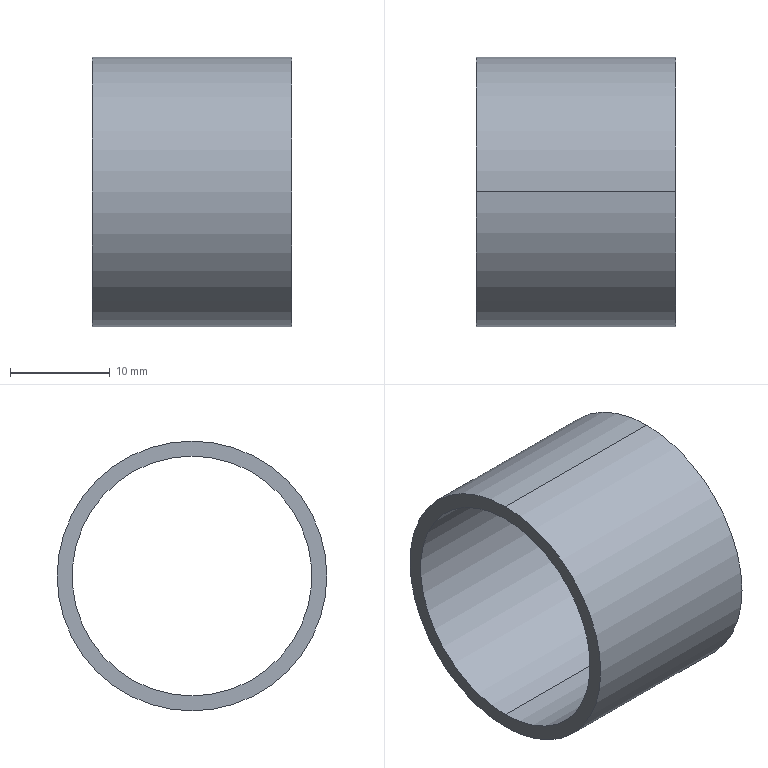Component | SolidWorks | ClampingAssembly-2_CopperSleeve24X27X10-2 | 1 solid | 6 faces | box 20 x 27 x 27 mm | volume 2403 mm3 | cylinder 4 | plane 2 | commonest cylinder face diameters 24 x2 27 x2 | material Bronze Bronze
build123d program:
from build123d import *

# Parameters (mm, degrees)
SKETCH1_R           = 13.5
SKETCH1_R_2         = 12
BOSS_EXTRUDE1_DEPTH = 20


with BuildPart() as part:
    # Sketch1 → Boss-Extrude1 (new body)
    with BuildSketch(Plane.XY):
        Circle(SKETCH1_R)
        Circle(SKETCH1_R_2, mode=Mode.SUBTRACT)
    extrude(amount=BOSS_EXTRUDE1_DEPTH)


solid = part.part

# Placed as in the assembly
solid = solid.moved(Location((-173.215, -74.917, -1210.457), (0, 90, 0)))
STEP:
#1=COLOUR_RGB('',0.7922,0.8196,0.9333);
#2=FILL_AREA_STYLE_COLOUR('',#1);
#3=FILL_AREA_STYLE('',(#2));
#4=SURFACE_STYLE_FILL_AREA(#3);
#5=SURFACE_SIDE_STYLE('',(#4));
#6=SURFACE_STYLE_USAGE(.BOTH.,#5);
#7=PRESENTATION_STYLE_ASSIGNMENT((#6));
#8=CARTESIAN_POINT('',(-6.819,-2.949,-47.183));
#9=VERTEX_POINT('',#8);
#10=CARTESIAN_POINT('',(-6.819,-2.949,-48.128));
#11=VERTEX_POINT('',#10);
#12=CARTESIAN_POINT('',(-6.819,-2.949,-47.656));
#13=DIRECTION('',(-1.,0.,-0.));
#14=DIRECTION('',(0.,0.,-1.));
#15=AXIS2_PLACEMENT_3D('',#12,#13,#14);
#16=CIRCLE('',#15,0.4724);
#17=EDGE_CURVE('',#9,#11,#16,.T.);
#18=ORIENTED_EDGE('',*,*,#17,.T.);
#19=CARTESIAN_POINT('',(-6.032,-2.949,-48.128));
#20=VERTEX_POINT('',#19);
#21=CARTESIAN_POINT('',(-6.819,-2.949,-48.128));
#22=DIRECTION('',(1.,-0.,0.));
#23=VECTOR('',#22,39.37);
#24=LINE('',#21,#23);
#25=EDGE_CURVE('',#11,#20,#24,.T.);
#26=ORIENTED_EDGE('',*,*,#25,.T.);
#27=CARTESIAN_POINT('',(-6.032,-2.949,-47.183));
#28=VERTEX_POINT('',#27);
#29=CARTESIAN_POINT('',(-6.032,-2.949,-47.656));
#30=DIRECTION('',(-1.,0.,-0.));
#31=DIRECTION('',(0.,0.,-1.));
#32=AXIS2_PLACEMENT_3D('',#29,#30,#31);
#33=CIRCLE('',#32,0.4724);
#34=EDGE_CURVE('',#28,#20,#33,.T.);
#35=ORIENTED_EDGE('',*,*,#34,.F.);
#36=CARTESIAN_POINT('',(-6.819,-2.949,-47.183));
#37=DIRECTION('',(1.,-0.,0.));
#38=VECTOR('',#37,39.37);
#39=LINE('',#36,#38);
#40=EDGE_CURVE('',#9,#28,#39,.T.);
#41=ORIENTED_EDGE('',*,*,#40,.F.);
#42=EDGE_LOOP('',(#18,#26,#35,#41));
#43=FACE_OUTER_BOUND('',#42,.T.);
#44=CARTESIAN_POINT('',(-6.819,-2.949,-47.656));
#45=DIRECTION('',(1.,-0.,0.));
#46=DIRECTION('',(0.,-0.,1.));
#47=AXIS2_PLACEMENT_3D('',#44,#45,#46);
#48=CYLINDRICAL_SURFACE('',#47,0.4724);
#49=ADVANCED_FACE('',(#43),#48,.F.);
#50=CARTESIAN_POINT('',(-6.819,-2.949,-48.187));
#51=VERTEX_POINT('',#50);
#52=CARTESIAN_POINT('',(-6.819,-2.949,-47.124));
#53=VERTEX_POINT('',#52);
#54=CARTESIAN_POINT('',(-6.819,-2.949,-47.656));
#55=DIRECTION('',(-1.,0.,-0.));
#56=DIRECTION('',(0.,0.,-1.));
#57=AXIS2_PLACEMENT_3D('',#54,#55,#56);
#58=CIRCLE('',#57,0.5315);
#59=EDGE_CURVE('',#51,#53,#58,.T.);
#60=ORIENTED_EDGE('',*,*,#59,.F.);
#61=CARTESIAN_POINT('',(-6.032,-2.949,-48.187));
#62=VERTEX_POINT('',#61);
#63=CARTESIAN_POINT('',(-6.819,-2.949,-48.187));
#64=DIRECTION('',(1.,-0.,0.));
#65=VECTOR('',#64,39.37);
#66=LINE('',#63,#65);
#67=EDGE_CURVE('',#51,#62,#66,.T.);
#68=ORIENTED_EDGE('',*,*,#67,.T.);
#69=CARTESIAN_POINT('',(-6.032,-2.949,-47.124));
#70=VERTEX_POINT('',#69);
#71=CARTESIAN_POINT('',(-6.032,-2.949,-47.656));
#72=DIRECTION('',(-1.,0.,-0.));
#73=DIRECTION('',(0.,0.,-1.));
#74=AXIS2_PLACEMENT_3D('',#71,#72,#73);
#75=CIRCLE('',#74,0.5315);
#76=EDGE_CURVE('',#62,#70,#75,.T.);
#77=ORIENTED_EDGE('',*,*,#76,.T.);
#78=CARTESIAN_POINT('',(-6.819,-2.949,-47.124));
#79=DIRECTION('',(1.,-0.,0.));
#80=VECTOR('',#79,39.37);
#81=LINE('',#78,#80);
#82=EDGE_CURVE('',#53,#70,#81,.T.);
#83=ORIENTED_EDGE('',*,*,#82,.F.);
#84=EDGE_LOOP('',(#60,#68,#77,#83));
#85=FACE_OUTER_BOUND('',#84,.T.);
#86=CARTESIAN_POINT('',(-6.819,-2.949,-47.656));
#87=DIRECTION('',(1.,-0.,0.));
#88=DIRECTION('',(0.,-0.,1.));
#89=AXIS2_PLACEMENT_3D('',#86,#87,#88);
#90=CYLINDRICAL_SURFACE('',#89,0.5315);
#91=ADVANCED_FACE('',(#85),#90,.T.);
#92=CARTESIAN_POINT('',(-6.819,-2.949,-47.656));
#93=DIRECTION('',(-1.,0.,-0.));
#94=DIRECTION('',(0.,0.,-1.));
#95=AXIS2_PLACEMENT_3D('',#92,#93,#94);
#96=CIRCLE('',#95,0.5315);
#97=EDGE_CURVE('',#53,#51,#96,.T.);
#98=ORIENTED_EDGE('',*,*,#97,.T.);
#99=ORIENTED_EDGE('',*,*,#59,.T.);
#100=EDGE_LOOP('',(#98,#99));
#101=FACE_OUTER_BOUND('',#100,.T.);
#102=ORIENTED_EDGE('',*,*,#17,.F.);
#103=CARTESIAN_POINT('',(-6.819,-2.949,-47.656));
#104=DIRECTION('',(-1.,0.,-0.));
#105=DIRECTION('',(0.,0.,-1.));
#106=AXIS2_PLACEMENT_3D('',#103,#104,#105);
#107=CIRCLE('',#106,0.4724);
#108=EDGE_CURVE('',#11,#9,#107,.T.);
#109=ORIENTED_EDGE('',*,*,#108,.F.);
#110=EDGE_LOOP('',(#102,#109));
#111=FACE_BOUND('',#110,.T.);
#112=CARTESIAN_POINT('',(-6.819,-2.949,-47.656));
#113=DIRECTION('',(-1.,0.,-0.));
#114=DIRECTION('',(0.,0.,-1.));
#115=AXIS2_PLACEMENT_3D('',#112,#113,#114);
#116=PLANE('',#115);
#117=ADVANCED_FACE('',(#101,#111),#116,.T.);
#118=CARTESIAN_POINT('',(-6.032,-2.949,-47.656));
#119=DIRECTION('',(-1.,0.,-0.));
#120=DIRECTION('',(0.,0.,-1.));
#121=AXIS2_PLACEMENT_3D('',#118,#119,#120);
#122=CIRCLE('',#121,0.5315);
#123=EDGE_CURVE('',#70,#62,#122,.T.);
#124=ORIENTED_EDGE('',*,*,#123,.F.);
#125=ORIENTED_EDGE('',*,*,#76,.F.);
#126=EDGE_LOOP('',(#124,#125));
#127=FACE_OUTER_BOUND('',#126,.T.);
#128=ORIENTED_EDGE('',*,*,#34,.T.);
#129=CARTESIAN_POINT('',(-6.032,-2.949,-47.656));
#130=DIRECTION('',(-1.,0.,-0.));
#131=DIRECTION('',(0.,0.,-1.));
#132=AXIS2_PLACEMENT_3D('',#129,#130,#131);
#133=CIRCLE('',#132,0.4724);
#134=EDGE_CURVE('',#20,#28,#133,.T.);
#135=ORIENTED_EDGE('',*,*,#134,.T.);
#136=EDGE_LOOP('',(#128,#135));
#137=FACE_BOUND('',#136,.T.);
#138=CARTESIAN_POINT('',(-6.032,-2.949,-47.656));
#139=DIRECTION('',(-1.,0.,-0.));
#140=DIRECTION('',(0.,0.,-1.));
#141=AXIS2_PLACEMENT_3D('',#138,#139,#140);
#142=PLANE('',#141);
#143=ADVANCED_FACE('',(#127,#137),#142,.F.);
#144=ORIENTED_EDGE('',*,*,#67,.F.);
#145=ORIENTED_EDGE('',*,*,#97,.F.);
#146=ORIENTED_EDGE('',*,*,#82,.T.);
#147=ORIENTED_EDGE('',*,*,#123,.T.);
#148=EDGE_LOOP('',(#144,#145,#146,#147));
#149=FACE_OUTER_BOUND('',#148,.T.);
#150=CARTESIAN_POINT('',(-6.819,-2.949,-47.656));
#151=DIRECTION('',(1.,-0.,0.));
#152=DIRECTION('',(0.,-0.,1.));
#153=AXIS2_PLACEMENT_3D('',#150,#151,#152);
#154=CYLINDRICAL_SURFACE('',#153,0.5315);
#155=ADVANCED_FACE('',(#149),#154,.T.);
#156=ORIENTED_EDGE('',*,*,#25,.F.);
#157=ORIENTED_EDGE('',*,*,#108,.T.);
#158=ORIENTED_EDGE('',*,*,#40,.T.);
#159=ORIENTED_EDGE('',*,*,#134,.F.);
#160=EDGE_LOOP('',(#156,#157,#158,#159));
#161=FACE_OUTER_BOUND('',#160,.T.);
#162=CARTESIAN_POINT('',(-6.819,-2.949,-47.656));
#163=DIRECTION('',(1.,-0.,0.));
#164=DIRECTION('',(0.,-0.,1.));
#165=AXIS2_PLACEMENT_3D('',#162,#163,#164);
#166=CYLINDRICAL_SURFACE('',#165,0.4724);
#167=ADVANCED_FACE('',(#161),#166,.F.);
#168=CLOSED_SHELL('',(#49,#91,#117,#143,#155,#167));
#169=MANIFOLD_SOLID_BREP('',#168);
#170=STYLED_ITEM('',(#7),#169);
#171=(LENGTH_UNIT()NAMED_UNIT(*)SI_UNIT($,.METRE.));
#172=LENGTH_MEASURE_WITH_UNIT(LENGTH_MEASURE(0.0254),#171);
#173=DIMENSIONAL_EXPONENTS(1.,0.,0.,0.,0.,0.,0.);
#174=(CONVERSION_BASED_UNIT('',#172)LENGTH_UNIT()NAMED_UNIT(#173));
#175=UNCERTAINTY_MEASURE_WITH_UNIT(LENGTH_MEASURE(0.00001),#174,'','');
#176=(NAMED_UNIT(*)PLANE_ANGLE_UNIT()SI_UNIT($,.RADIAN.));
#177=(NAMED_UNIT(*)SI_UNIT($,.STERADIAN.)SOLID_ANGLE_UNIT());
#178=(GEOMETRIC_REPRESENTATION_CONTEXT(3)GLOBAL_UNCERTAINTY_ASSIGNED_CONTEXT((#175))GLOBAL_UNIT_ASSIGNED_CONTEXT((#174,#176,#177))REPRESENTATION_CONTEXT('',''));
#179=MECHANICAL_DESIGN_GEOMETRIC_PRESENTATION_REPRESENTATION('',(#170),#178);
#180=CARTESIAN_POINT('',(0.,0.,0.));
#181=DIRECTION('',(0.,0.,1.));
#182=DIRECTION('',(1.,0.,0.));
#183=AXIS2_PLACEMENT_3D('',#180,#181,#182);
#184=(LENGTH_UNIT()NAMED_UNIT(*)SI_UNIT($,.METRE.));
#185=LENGTH_MEASURE_WITH_UNIT(LENGTH_MEASURE(0.0254),#184);
#186=DIMENSIONAL_EXPONENTS(1.,0.,0.,0.,0.,0.,0.);
#187=(CONVERSION_BASED_UNIT('',#185)LENGTH_UNIT()NAMED_UNIT(#186));
#188=UNCERTAINTY_MEASURE_WITH_UNIT(LENGTH_MEASURE(0.00001),#187,'','');
#189=(NAMED_UNIT(*)PLANE_ANGLE_UNIT()SI_UNIT($,.RADIAN.));
#190=(NAMED_UNIT(*)SI_UNIT($,.STERADIAN.)SOLID_ANGLE_UNIT());
#191=(GEOMETRIC_REPRESENTATION_CONTEXT(3)GLOBAL_UNCERTAINTY_ASSIGNED_CONTEXT((#188))GLOBAL_UNIT_ASSIGNED_CONTEXT((#187,#189,#190))REPRESENTATION_CONTEXT('',''));
#192=ADVANCED_BREP_SHAPE_REPRESENTATION('',(#169,#183),#191);
#193=PRESENTATION_LAYER_ASSIGNMENT('','',(#170));